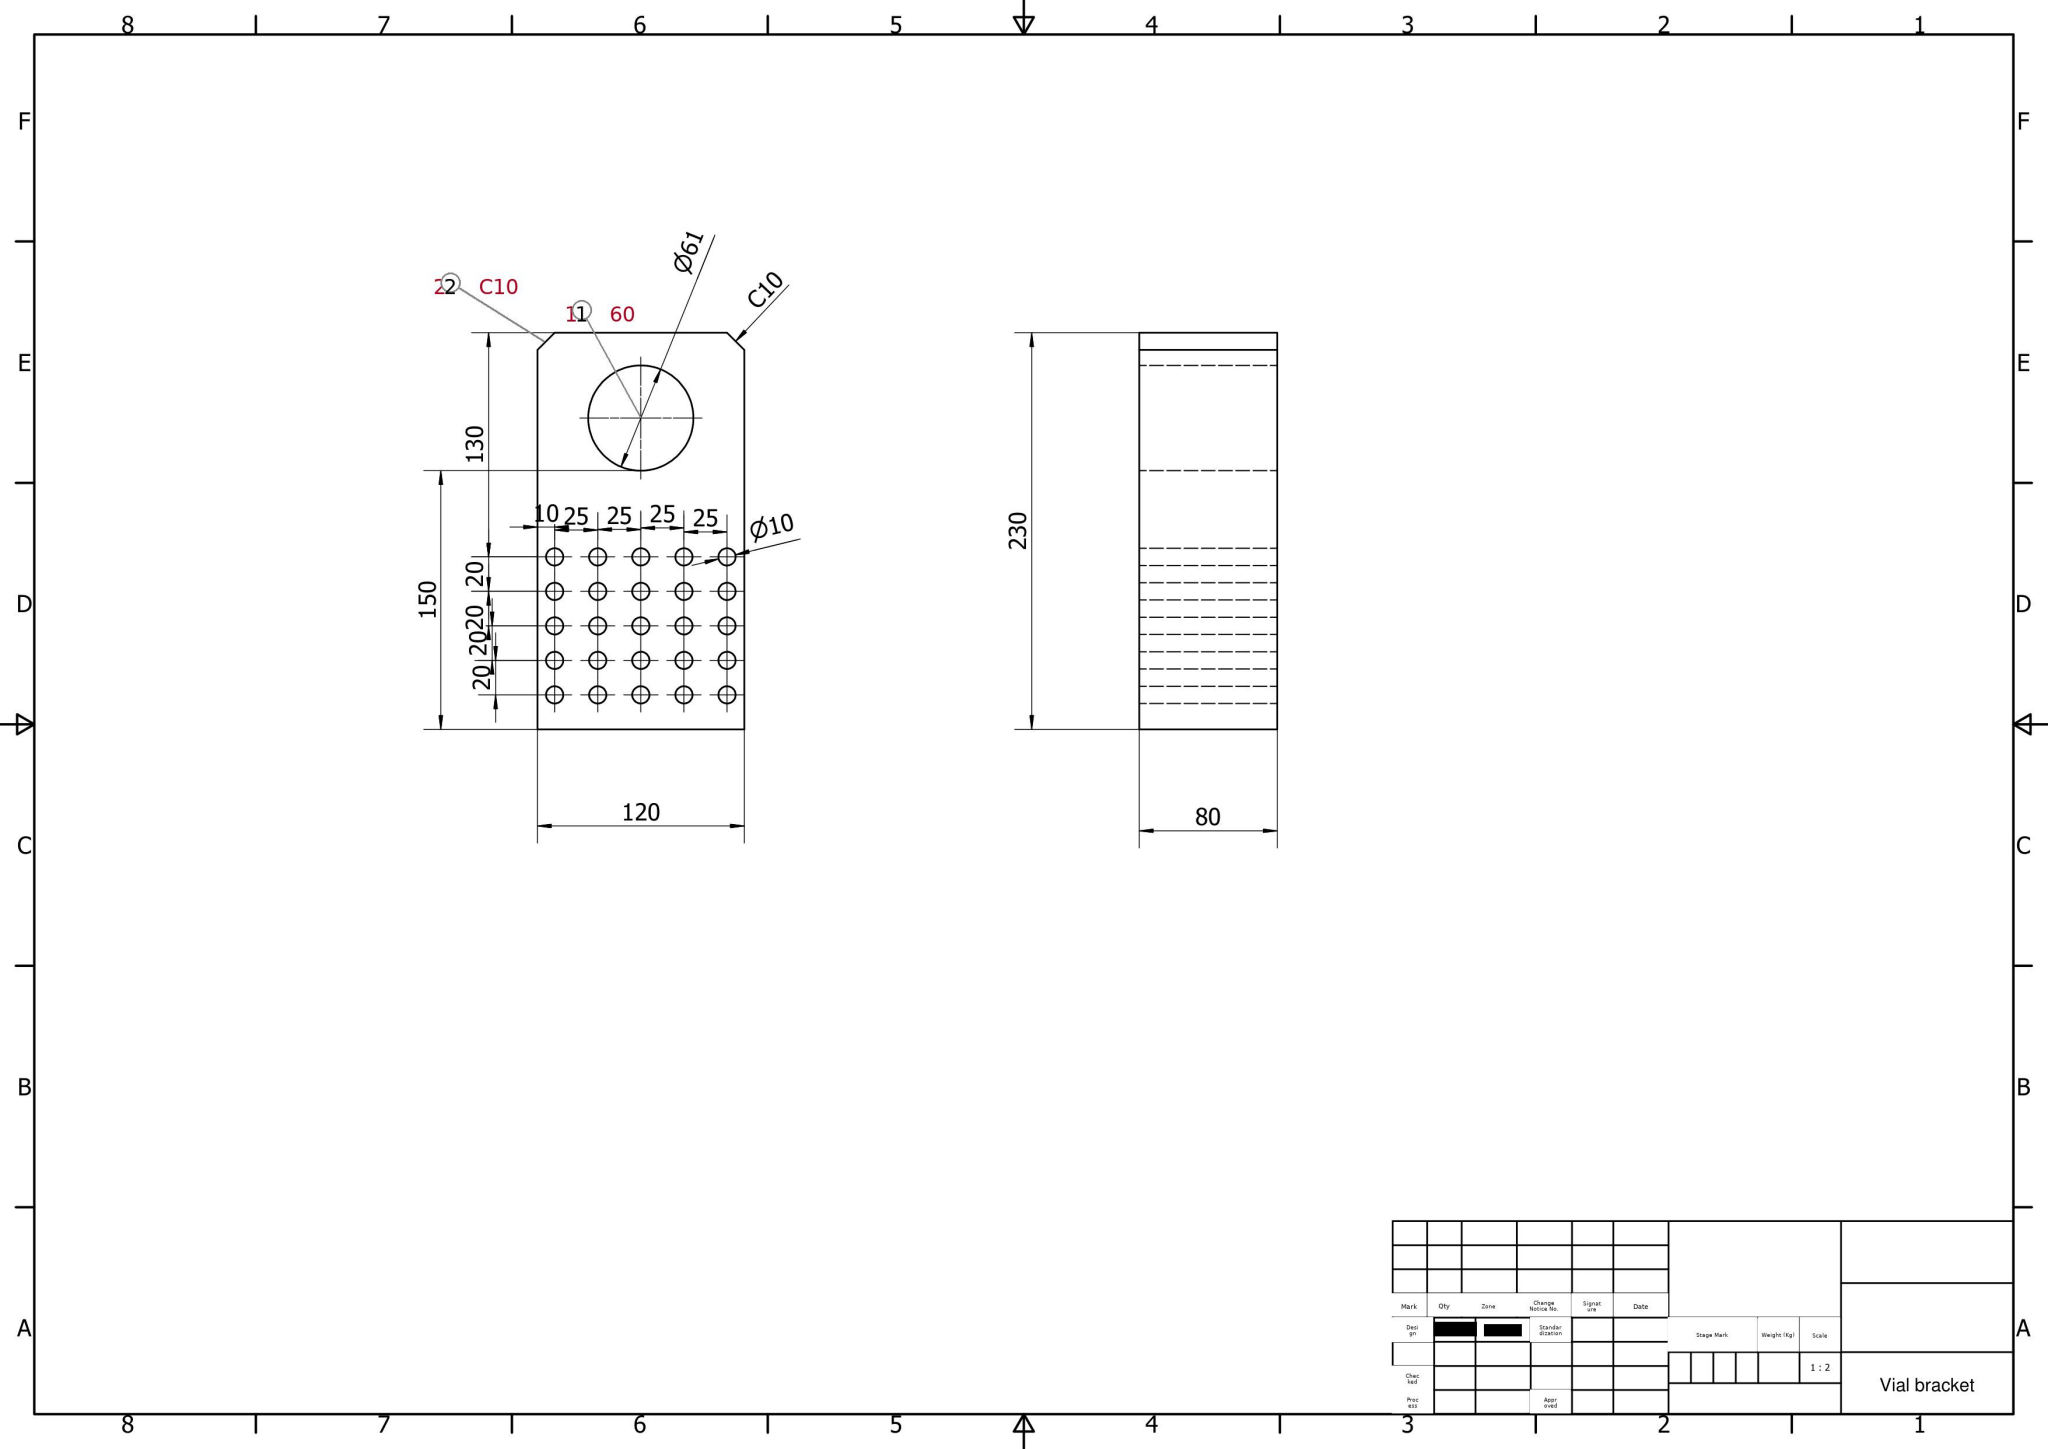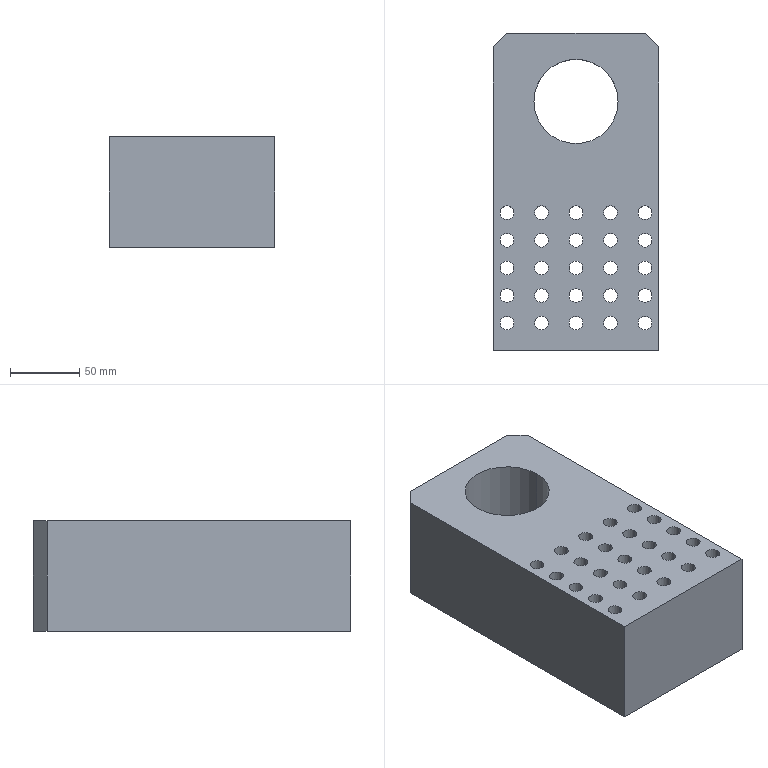Part | SolidWorks | mm | 1 solid | 60 faces | box 120 x 230 x 80 mm | volume 1809123 mm3 | cylinder 52 | plane 8 | commonest cylinder face diameters 10 x50 61 x2